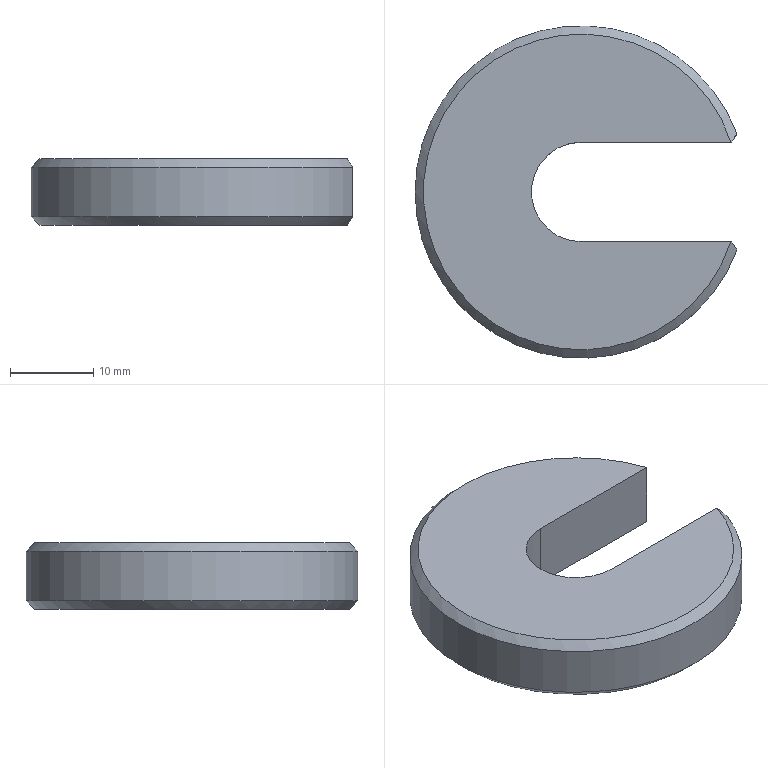Component | NX | SPLIT_WASHER | 1 solid | 10 faces | box 38.74 x 40 x 8 mm | volume 7592 mm3 | plane 6 | cylinder 2 | cone 2 | commonest cylinder face diameters 40 x1 12 x1
STEP:
#1=CARTESIAN_POINT('',(0.,0.,0.));
#2=DIRECTION('',(0.,0.,1.));
#3=DIRECTION('',(1.,0.,0.));
#4=AXIS2_PLACEMENT_3D('',#1,#2,#3);
#5=CARTESIAN_POINT('',(108.735,77.382,82.));
#6=VERTEX_POINT('',#5);
#7=CARTESIAN_POINT('',(108.735,77.382,76.));
#8=VERTEX_POINT('',#7);
#9=CARTESIAN_POINT('',(108.735,77.382,83.));
#10=DIRECTION('',(0.,0.,-1.));
#11=VECTOR('',#10,1.);
#12=LINE('',#9,#11);
#13=CARTESIAN_POINT('',(89.996,70.391,83.));
#14=DIRECTION('',(0.,0.,-1.));
#15=DIRECTION('',(-1.,0.,0.));
#16=AXIS2_PLACEMENT_3D('',#13,#14,#15);
#17=CYLINDRICAL_SURFACE('',#16,20.);
#18=CARTESIAN_POINT('',(2.785,0.));
#19=DIRECTION('',(0.,1.));
#20=VECTOR('',#19,1.);
#21=LINE('',#18,#20);
#22=(GEOMETRIC_REPRESENTATION_CONTEXT(2)PARAMETRIC_REPRESENTATION_CONTEXT()REPRESENTATION_CONTEXT('',''));
#23=DEFINITIONAL_REPRESENTATION('',(#21),#22);
#24=PCURVE('',#17,#23);
#25=CARTESIAN_POINT('',(108.735,77.382,83.));
#26=DIRECTION('',(-0.8214,0.5703,0.));
#27=DIRECTION('',(0.,0.,-1.));
#28=AXIS2_PLACEMENT_3D('',#25,#26,#27);
#29=PLANE('',#28);
#30=CARTESIAN_POINT('',(0.,0.));
#31=DIRECTION('',(1.,0.));
#32=VECTOR('',#31,1.);
#33=LINE('',#30,#32);
#34=(GEOMETRIC_REPRESENTATION_CONTEXT(2)PARAMETRIC_REPRESENTATION_CONTEXT()REPRESENTATION_CONTEXT('',''));
#35=DEFINITIONAL_REPRESENTATION('',(#33),#34);
#36=PCURVE('',#29,#35);
#37=SURFACE_CURVE('',#12,(#24,#36),.PCURVE_S1.);
#38=EDGE_CURVE('',#6,#8,#37,.T.);
#39=ORIENTED_EDGE('',*,*,#38,.T.);
#40=CARTESIAN_POINT('',(108.735,63.401,76.));
#41=VERTEX_POINT('',#40);
#42=CARTESIAN_POINT('',(89.996,70.391,76.));
#43=DIRECTION('',(0.,0.,1.));
#44=DIRECTION('',(1.,0.,0.));
#45=AXIS2_PLACEMENT_3D('',#42,#43,#44);
#46=CIRCLE('',#45,20.);
#47=CARTESIAN_POINT('',(3.142,7.));
#48=DIRECTION('',(-1.,0.));
#49=VECTOR('',#48,1.);
#50=LINE('',#47,#49);
#51=(GEOMETRIC_REPRESENTATION_CONTEXT(2)PARAMETRIC_REPRESENTATION_CONTEXT()REPRESENTATION_CONTEXT('',''));
#52=DEFINITIONAL_REPRESENTATION('',(#50),#51);
#53=PCURVE('',#17,#52);
#54=CARTESIAN_POINT('',(89.996,70.391,76.));
#55=DIRECTION('',(0.,0.,1.));
#56=DIRECTION('',(1.,0.,0.));
#57=AXIS2_PLACEMENT_3D('',#54,#55,#56);
#58=CONICAL_SURFACE('',#57,20.,0.7854);
#59=CARTESIAN_POINT('',(-0.,-0.));
#60=DIRECTION('',(1.,0.));
#61=VECTOR('',#60,1.);
#62=LINE('',#59,#61);
#63=(GEOMETRIC_REPRESENTATION_CONTEXT(2)PARAMETRIC_REPRESENTATION_CONTEXT()REPRESENTATION_CONTEXT('',''));
#64=DEFINITIONAL_REPRESENTATION('',(#62),#63);
#65=PCURVE('',#58,#64);
#66=SURFACE_CURVE('',#46,(#53,#65),.PCURVE_S1.);
#67=EDGE_CURVE('',#8,#41,#66,.T.);
#68=ORIENTED_EDGE('',*,*,#67,.T.);
#69=CARTESIAN_POINT('',(108.735,63.401,82.));
#70=VERTEX_POINT('',#69);
#71=CARTESIAN_POINT('',(108.735,63.401,83.));
#72=DIRECTION('',(0.,0.,1.));
#73=VECTOR('',#72,1.);
#74=LINE('',#71,#73);
#75=CARTESIAN_POINT('',(-2.785,0.));
#76=DIRECTION('',(0.,-1.));
#77=VECTOR('',#76,1.);
#78=LINE('',#75,#77);
#79=(GEOMETRIC_REPRESENTATION_CONTEXT(2)PARAMETRIC_REPRESENTATION_CONTEXT()REPRESENTATION_CONTEXT('',''));
#80=DEFINITIONAL_REPRESENTATION('',(#78),#79);
#81=PCURVE('',#17,#80);
#82=CARTESIAN_POINT('',(108.047,64.391,83.));
#83=DIRECTION('',(-0.8214,-0.5703,0.));
#84=DIRECTION('',(0.,0.,-1.));
#85=AXIS2_PLACEMENT_3D('',#82,#83,#84);
#86=PLANE('',#85);
#87=CARTESIAN_POINT('',(0.,1.206));
#88=DIRECTION('',(-1.,0.));
#89=VECTOR('',#88,1.);
#90=LINE('',#87,#89);
#91=(GEOMETRIC_REPRESENTATION_CONTEXT(2)PARAMETRIC_REPRESENTATION_CONTEXT()REPRESENTATION_CONTEXT('',''));
#92=DEFINITIONAL_REPRESENTATION('',(#90),#91);
#93=PCURVE('',#86,#92);
#94=SURFACE_CURVE('',#74,(#81,#93),.PCURVE_S1.);
#95=EDGE_CURVE('',#41,#70,#94,.T.);
#96=ORIENTED_EDGE('',*,*,#95,.T.);
#97=CARTESIAN_POINT('',(89.996,70.391,82.));
#98=DIRECTION('',(0.,0.,-1.));
#99=DIRECTION('',(1.,0.,0.));
#100=AXIS2_PLACEMENT_3D('',#97,#98,#99);
#101=CIRCLE('',#100,20.);
#102=CARTESIAN_POINT('',(-3.142,1.));
#103=DIRECTION('',(1.,0.));
#104=VECTOR('',#103,1.);
#105=LINE('',#102,#104);
#106=(GEOMETRIC_REPRESENTATION_CONTEXT(2)PARAMETRIC_REPRESENTATION_CONTEXT()REPRESENTATION_CONTEXT('',''));
#107=DEFINITIONAL_REPRESENTATION('',(#105),#106);
#108=PCURVE('',#17,#107);
#109=CARTESIAN_POINT('',(89.996,70.391,83.));
#110=DIRECTION('',(0.,0.,-1.));
#111=DIRECTION('',(-1.,0.,0.));
#112=AXIS2_PLACEMENT_3D('',#109,#110,#111);
#113=CONICAL_SURFACE('',#112,19.,0.7854);
#114=CARTESIAN_POINT('',(-3.142,1.));
#115=DIRECTION('',(1.,0.));
#116=VECTOR('',#115,1.);
#117=LINE('',#114,#116);
#118=(GEOMETRIC_REPRESENTATION_CONTEXT(2)PARAMETRIC_REPRESENTATION_CONTEXT()REPRESENTATION_CONTEXT('',''));
#119=DEFINITIONAL_REPRESENTATION('',(#117),#118);
#120=PCURVE('',#113,#119);
#121=SURFACE_CURVE('',#101,(#108,#120),.PCURVE_S1.);
#122=EDGE_CURVE('',#70,#6,#121,.T.);
#123=ORIENTED_EDGE('',*,*,#122,.T.);
#124=EDGE_LOOP('',(#39,#68,#96,#123));
#125=FACE_BOUND('',#124,.T.);
#126=ADVANCED_FACE('',(#125),#17,.T.);
#127=CARTESIAN_POINT('',(108.047,64.391,82.978));
#128=VERTEX_POINT('',#127);
#129=CARTESIAN_POINT('',(108.047,64.391,75.022));
#130=VERTEX_POINT('',#129);
#131=CARTESIAN_POINT('',(108.047,64.391,83.));
#132=DIRECTION('',(0.,0.,-1.));
#133=VECTOR('',#132,1.);
#134=LINE('',#131,#133);
#135=CARTESIAN_POINT('',(109.075,64.391,83.));
#136=DIRECTION('',(0.,-1.,0.));
#137=DIRECTION('',(0.,0.,-1.));
#138=AXIS2_PLACEMENT_3D('',#135,#136,#137);
#139=PLANE('',#138);
#140=CARTESIAN_POINT('',(0.,-1.028));
#141=DIRECTION('',(1.,0.));
#142=VECTOR('',#141,1.);
#143=LINE('',#140,#142);
#144=(GEOMETRIC_REPRESENTATION_CONTEXT(2)PARAMETRIC_REPRESENTATION_CONTEXT()REPRESENTATION_CONTEXT('',''));
#145=DEFINITIONAL_REPRESENTATION('',(#143),#144);
#146=PCURVE('',#139,#145);
#147=CARTESIAN_POINT('',(0.,0.));
#148=DIRECTION('',(1.,0.));
#149=VECTOR('',#148,1.);
#150=LINE('',#147,#149);
#151=(GEOMETRIC_REPRESENTATION_CONTEXT(2)PARAMETRIC_REPRESENTATION_CONTEXT()REPRESENTATION_CONTEXT('',''));
#152=DEFINITIONAL_REPRESENTATION('',(#150),#151);
#153=PCURVE('',#86,#152);
#154=SURFACE_CURVE('',#134,(#146,#153),.PCURVE_S1.);
#155=EDGE_CURVE('',#128,#130,#154,.T.);
#156=ORIENTED_EDGE('',*,*,#155,.T.);
#157=CARTESIAN_POINT('',(108.024,64.391,75.));
#158=VERTEX_POINT('',#157);
#159=CARTESIAN_POINT('',(108.047,64.391,75.022));
#160=CARTESIAN_POINT('',(108.039,64.391,75.015));
#161=CARTESIAN_POINT('',(108.031,64.391,75.007));
#162=CARTESIAN_POINT('',(108.024,64.391,75.));
#163=B_SPLINE_CURVE_WITH_KNOTS('',3,(#159,#160,#161,#162),.UNSPECIFIED.,.F.,.F.,(4,4),(0.,1.),.PIECEWISE_BEZIER_KNOTS.);
#164=CARTESIAN_POINT('',(7.978,-1.028));
#165=CARTESIAN_POINT('',(7.985,-1.035));
#166=CARTESIAN_POINT('',(7.993,-1.043));
#167=CARTESIAN_POINT('',(8.,-1.051));
#168=B_SPLINE_CURVE_WITH_KNOTS('',3,(#164,#165,#166,#167),.UNSPECIFIED.,.F.,.F.,(4,4),(0.,1.),.PIECEWISE_BEZIER_KNOTS.);
#169=(GEOMETRIC_REPRESENTATION_CONTEXT(2)PARAMETRIC_REPRESENTATION_CONTEXT()REPRESENTATION_CONTEXT('',''));
#170=DEFINITIONAL_REPRESENTATION('',(#168),#169);
#171=PCURVE('',#139,#170);
#172=CARTESIAN_POINT('',(5.962,-0.9778));
#173=CARTESIAN_POINT('',(5.962,-1.));
#174=B_SPLINE_CURVE_WITH_KNOTS('',1,(#172,#173),.UNSPECIFIED.,.F.,.F.,(2,2),(0.,1.),.PIECEWISE_BEZIER_KNOTS.);
#175=(GEOMETRIC_REPRESENTATION_CONTEXT(2)PARAMETRIC_REPRESENTATION_CONTEXT()REPRESENTATION_CONTEXT('',''));
#176=DEFINITIONAL_REPRESENTATION('',(#174),#175);
#177=PCURVE('',#58,#176);
#178=SURFACE_CURVE('',#163,(#171,#177),.PCURVE_S1.);
#179=EDGE_CURVE('',#130,#158,#178,.T.);
#180=ORIENTED_EDGE('',*,*,#179,.T.);
#181=CARTESIAN_POINT('',(89.996,64.391,75.));
#182=VERTEX_POINT('',#181);
#183=CARTESIAN_POINT('',(109.075,64.391,75.));
#184=DIRECTION('',(-1.,0.,0.));
#185=VECTOR('',#184,1.);
#186=LINE('',#183,#185);
#187=CARTESIAN_POINT('',(8.,0.));
#188=DIRECTION('',(0.,-1.));
#189=VECTOR('',#188,1.);
#190=LINE('',#187,#189);
#191=(GEOMETRIC_REPRESENTATION_CONTEXT(2)PARAMETRIC_REPRESENTATION_CONTEXT()REPRESENTATION_CONTEXT('',''));
#192=DEFINITIONAL_REPRESENTATION('',(#190),#191);
#193=PCURVE('',#139,#192);
#194=CARTESIAN_POINT('',(89.996,70.391,75.));
#195=DIRECTION('',(0.,0.,1.));
#196=DIRECTION('',(1.,0.,0.));
#197=AXIS2_PLACEMENT_3D('',#194,#195,#196);
#198=PLANE('',#197);
#199=CARTESIAN_POINT('',(19.079,-6.));
#200=DIRECTION('',(-1.,0.));
#201=VECTOR('',#200,1.);
#202=LINE('',#199,#201);
#203=(GEOMETRIC_REPRESENTATION_CONTEXT(2)PARAMETRIC_REPRESENTATION_CONTEXT()REPRESENTATION_CONTEXT('',''));
#204=DEFINITIONAL_REPRESENTATION('',(#202),#203);
#205=PCURVE('',#198,#204);
#206=SURFACE_CURVE('',#186,(#193,#205),.PCURVE_S1.);
#207=EDGE_CURVE('',#158,#182,#206,.T.);
#208=ORIENTED_EDGE('',*,*,#207,.T.);
#209=CARTESIAN_POINT('',(89.996,64.391,83.));
#210=VERTEX_POINT('',#209);
#211=CARTESIAN_POINT('',(89.996,64.391,83.));
#212=DIRECTION('',(0.,0.,-1.));
#213=VECTOR('',#212,1.);
#214=LINE('',#211,#213);
#215=CARTESIAN_POINT('',(0.,-19.079));
#216=DIRECTION('',(1.,0.));
#217=VECTOR('',#216,1.);
#218=LINE('',#215,#217);
#219=(GEOMETRIC_REPRESENTATION_CONTEXT(2)PARAMETRIC_REPRESENTATION_CONTEXT()REPRESENTATION_CONTEXT('',''));
#220=DEFINITIONAL_REPRESENTATION('',(#218),#219);
#221=PCURVE('',#139,#220);
#222=CARTESIAN_POINT('',(89.996,70.391,83.));
#223=DIRECTION('',(0.,0.,-1.));
#224=DIRECTION('',(-1.,0.,0.));
#225=AXIS2_PLACEMENT_3D('',#222,#223,#224);
#226=CYLINDRICAL_SURFACE('',#225,6.);
#227=CARTESIAN_POINT('',(-1.571,0.));
#228=DIRECTION('',(0.,1.));
#229=VECTOR('',#228,1.);
#230=LINE('',#227,#229);
#231=(GEOMETRIC_REPRESENTATION_CONTEXT(2)PARAMETRIC_REPRESENTATION_CONTEXT()REPRESENTATION_CONTEXT('',''));
#232=DEFINITIONAL_REPRESENTATION('',(#230),#231);
#233=PCURVE('',#226,#232);
#234=SURFACE_CURVE('',#214,(#221,#233),.PCURVE_S1.);
#235=EDGE_CURVE('',#210,#182,#234,.T.);
#236=ORIENTED_EDGE('',*,*,#235,.F.);
#237=CARTESIAN_POINT('',(108.024,64.391,83.));
#238=VERTEX_POINT('',#237);
#239=CARTESIAN_POINT('',(109.075,64.391,83.));
#240=DIRECTION('',(-1.,0.,0.));
#241=VECTOR('',#240,1.);
#242=LINE('',#239,#241);
#243=CARTESIAN_POINT('',(0.,0.));
#244=DIRECTION('',(0.,-1.));
#245=VECTOR('',#244,1.);
#246=LINE('',#243,#245);
#247=(GEOMETRIC_REPRESENTATION_CONTEXT(2)PARAMETRIC_REPRESENTATION_CONTEXT()REPRESENTATION_CONTEXT('',''));
#248=DEFINITIONAL_REPRESENTATION('',(#246),#247);
#249=PCURVE('',#139,#248);
#250=CARTESIAN_POINT('',(89.996,70.391,83.));
#251=DIRECTION('',(0.,0.,1.));
#252=DIRECTION('',(1.,0.,0.));
#253=AXIS2_PLACEMENT_3D('',#250,#251,#252);
#254=PLANE('',#253);
#255=CARTESIAN_POINT('',(19.079,-6.));
#256=DIRECTION('',(-1.,0.));
#257=VECTOR('',#256,1.);
#258=LINE('',#255,#257);
#259=(GEOMETRIC_REPRESENTATION_CONTEXT(2)PARAMETRIC_REPRESENTATION_CONTEXT()REPRESENTATION_CONTEXT('',''));
#260=DEFINITIONAL_REPRESENTATION('',(#258),#259);
#261=PCURVE('',#254,#260);
#262=SURFACE_CURVE('',#242,(#249,#261),.PCURVE_S1.);
#263=EDGE_CURVE('',#238,#210,#262,.T.);
#264=ORIENTED_EDGE('',*,*,#263,.F.);
#265=CARTESIAN_POINT('',(108.024,64.391,83.));
#266=CARTESIAN_POINT('',(108.031,64.391,82.993));
#267=CARTESIAN_POINT('',(108.039,64.391,82.985));
#268=CARTESIAN_POINT('',(108.047,64.391,82.978));
#269=B_SPLINE_CURVE_WITH_KNOTS('',3,(#265,#266,#267,#268),.UNSPECIFIED.,.F.,.F.,(4,4),(0.,1.),.PIECEWISE_BEZIER_KNOTS.);
#270=CARTESIAN_POINT('',(0.,-1.051));
#271=CARTESIAN_POINT('',(0.007385,-1.043));
#272=CARTESIAN_POINT('',(0.01477,-1.035));
#273=CARTESIAN_POINT('',(0.02216,-1.028));
#274=B_SPLINE_CURVE_WITH_KNOTS('',3,(#270,#271,#272,#273),.UNSPECIFIED.,.F.,.F.,(4,4),(0.,1.),.PIECEWISE_BEZIER_KNOTS.);
#275=(GEOMETRIC_REPRESENTATION_CONTEXT(2)PARAMETRIC_REPRESENTATION_CONTEXT()REPRESENTATION_CONTEXT('',''));
#276=DEFINITIONAL_REPRESENTATION('',(#274),#275);
#277=PCURVE('',#139,#276);
#278=CARTESIAN_POINT('',(-2.82,0.));
#279=CARTESIAN_POINT('',(-2.821,0.02216));
#280=B_SPLINE_CURVE_WITH_KNOTS('',1,(#278,#279),.UNSPECIFIED.,.F.,.F.,(2,2),(0.,1.),.PIECEWISE_BEZIER_KNOTS.);
#281=(GEOMETRIC_REPRESENTATION_CONTEXT(2)PARAMETRIC_REPRESENTATION_CONTEXT()REPRESENTATION_CONTEXT('',''));
#282=DEFINITIONAL_REPRESENTATION('',(#280),#281);
#283=PCURVE('',#113,#282);
#284=SURFACE_CURVE('',#269,(#277,#283),.PCURVE_S1.);
#285=EDGE_CURVE('',#238,#128,#284,.T.);
#286=ORIENTED_EDGE('',*,*,#285,.T.);
#287=EDGE_LOOP('',(#156,#180,#208,#236,#264,#286));
#288=FACE_BOUND('',#287,.T.);
#289=ADVANCED_FACE('',(#288),#139,.F.);
#290=ORIENTED_EDGE('',*,*,#235,.F.);
#291=CARTESIAN_POINT('',(89.996,76.391,83.));
#292=VERTEX_POINT('',#291);
#293=CARTESIAN_POINT('',(89.996,70.391,83.));
#294=DIRECTION('',(0.,0.,-1.));
#295=DIRECTION('',(1.,0.,0.));
#296=AXIS2_PLACEMENT_3D('',#293,#294,#295);
#297=CIRCLE('',#296,6.);
#298=CARTESIAN_POINT('',(-3.142,0.));
#299=DIRECTION('',(1.,0.));
#300=VECTOR('',#299,1.);
#301=LINE('',#298,#300);
#302=(GEOMETRIC_REPRESENTATION_CONTEXT(2)PARAMETRIC_REPRESENTATION_CONTEXT()REPRESENTATION_CONTEXT('',''));
#303=DEFINITIONAL_REPRESENTATION('',(#301),#302);
#304=PCURVE('',#226,#303);
#305=CARTESIAN_POINT('',(6.,0.));
#306=CARTESIAN_POINT('',(6.,-10.392));
#307=CARTESIAN_POINT('',(-3.,-5.196));
#308=CARTESIAN_POINT('',(-12.,-0.));
#309=CARTESIAN_POINT('',(-3.,5.196));
#310=CARTESIAN_POINT('',(6.,10.392));
#311=CARTESIAN_POINT('',(6.,0.));
#312=(BOUNDED_CURVE()B_SPLINE_CURVE(2,(#305,#306,#307,#308,#309,#310,#311),.UNSPECIFIED.,.T.,.F.)B_SPLINE_CURVE_WITH_KNOTS((1,2,2,2,2,1),(-2.094,0.,2.094,4.189,6.283,8.378),.UNSPECIFIED.)CURVE()GEOMETRIC_REPRESENTATION_ITEM()RATIONAL_B_SPLINE_CURVE((1.,0.5,1.,0.5,1.,0.5,1.))REPRESENTATION_ITEM(''));
#313=(GEOMETRIC_REPRESENTATION_CONTEXT(2)PARAMETRIC_REPRESENTATION_CONTEXT()REPRESENTATION_CONTEXT('',''));
#314=DEFINITIONAL_REPRESENTATION('',(#312),#313);
#315=PCURVE('',#254,#314);
#316=SURFACE_CURVE('',#297,(#304,#315),.PCURVE_S1.);
#317=EDGE_CURVE('',#210,#292,#316,.T.);
#318=ORIENTED_EDGE('',*,*,#317,.T.);
#319=CARTESIAN_POINT('',(89.996,76.391,75.));
#320=VERTEX_POINT('',#319);
#321=CARTESIAN_POINT('',(89.996,76.391,83.));
#322=DIRECTION('',(0.,0.,-1.));
#323=VECTOR('',#322,1.);
#324=LINE('',#321,#323);
#325=CARTESIAN_POINT('',(1.571,0.));
#326=DIRECTION('',(0.,1.));
#327=VECTOR('',#326,1.);
#328=LINE('',#325,#327);
#329=(GEOMETRIC_REPRESENTATION_CONTEXT(2)PARAMETRIC_REPRESENTATION_CONTEXT()REPRESENTATION_CONTEXT('',''));
#330=DEFINITIONAL_REPRESENTATION('',(#328),#329);
#331=PCURVE('',#226,#330);
#332=CARTESIAN_POINT('',(89.996,76.391,83.));
#333=DIRECTION('',(0.,1.,0.));
#334=DIRECTION('',(0.,0.,1.));
#335=AXIS2_PLACEMENT_3D('',#332,#333,#334);
#336=PLANE('',#335);
#337=CARTESIAN_POINT('',(0.,0.));
#338=DIRECTION('',(-1.,0.));
#339=VECTOR('',#338,1.);
#340=LINE('',#337,#339);
#341=(GEOMETRIC_REPRESENTATION_CONTEXT(2)PARAMETRIC_REPRESENTATION_CONTEXT()REPRESENTATION_CONTEXT('',''));
#342=DEFINITIONAL_REPRESENTATION('',(#340),#341);
#343=PCURVE('',#336,#342);
#344=SURFACE_CURVE('',#324,(#331,#343),.PCURVE_S1.);
#345=EDGE_CURVE('',#292,#320,#344,.T.);
#346=ORIENTED_EDGE('',*,*,#345,.T.);
#347=CARTESIAN_POINT('',(89.996,70.391,75.));
#348=DIRECTION('',(0.,0.,-1.));
#349=DIRECTION('',(1.,0.,0.));
#350=AXIS2_PLACEMENT_3D('',#347,#348,#349);
#351=CIRCLE('',#350,6.);
#352=CARTESIAN_POINT('',(-3.142,8.));
#353=DIRECTION('',(1.,0.));
#354=VECTOR('',#353,1.);
#355=LINE('',#352,#354);
#356=(GEOMETRIC_REPRESENTATION_CONTEXT(2)PARAMETRIC_REPRESENTATION_CONTEXT()REPRESENTATION_CONTEXT('',''));
#357=DEFINITIONAL_REPRESENTATION('',(#355),#356);
#358=PCURVE('',#226,#357);
#359=CARTESIAN_POINT('',(6.,0.));
#360=CARTESIAN_POINT('',(6.,-10.392));
#361=CARTESIAN_POINT('',(-3.,-5.196));
#362=CARTESIAN_POINT('',(-12.,-0.));
#363=CARTESIAN_POINT('',(-3.,5.196));
#364=CARTESIAN_POINT('',(6.,10.392));
#365=CARTESIAN_POINT('',(6.,0.));
#366=(BOUNDED_CURVE()B_SPLINE_CURVE(2,(#359,#360,#361,#362,#363,#364,#365),.UNSPECIFIED.,.T.,.F.)B_SPLINE_CURVE_WITH_KNOTS((1,2,2,2,2,1),(-2.094,0.,2.094,4.189,6.283,8.378),.UNSPECIFIED.)CURVE()GEOMETRIC_REPRESENTATION_ITEM()RATIONAL_B_SPLINE_CURVE((1.,0.5,1.,0.5,1.,0.5,1.))REPRESENTATION_ITEM(''));
#367=(GEOMETRIC_REPRESENTATION_CONTEXT(2)PARAMETRIC_REPRESENTATION_CONTEXT()REPRESENTATION_CONTEXT('',''));
#368=DEFINITIONAL_REPRESENTATION('',(#366),#367);
#369=PCURVE('',#198,#368);
#370=SURFACE_CURVE('',#351,(#358,#369),.PCURVE_S1.);
#371=EDGE_CURVE('',#182,#320,#370,.T.);
#372=ORIENTED_EDGE('',*,*,#371,.F.);
#373=EDGE_LOOP('',(#290,#318,#346,#372));
#374=FACE_BOUND('',#373,.F.);
#375=ADVANCED_FACE('',(#374),#226,.F.);
#376=CARTESIAN_POINT('',(108.024,76.391,75.));
#377=VERTEX_POINT('',#376);
#378=CARTESIAN_POINT('',(89.996,76.391,75.));
#379=DIRECTION('',(1.,0.,0.));
#380=VECTOR('',#379,1.);
#381=LINE('',#378,#380);
#382=CARTESIAN_POINT('',(-8.,0.));
#383=DIRECTION('',(0.,1.));
#384=VECTOR('',#383,1.);
#385=LINE('',#382,#384);
#386=(GEOMETRIC_REPRESENTATION_CONTEXT(2)PARAMETRIC_REPRESENTATION_CONTEXT()REPRESENTATION_CONTEXT('',''));
#387=DEFINITIONAL_REPRESENTATION('',(#385),#386);
#388=PCURVE('',#336,#387);
#389=CARTESIAN_POINT('',(0.,6.));
#390=DIRECTION('',(1.,0.));
#391=VECTOR('',#390,1.);
#392=LINE('',#389,#391);
#393=(GEOMETRIC_REPRESENTATION_CONTEXT(2)PARAMETRIC_REPRESENTATION_CONTEXT()REPRESENTATION_CONTEXT('',''));
#394=DEFINITIONAL_REPRESENTATION('',(#392),#393);
#395=PCURVE('',#198,#394);
#396=SURFACE_CURVE('',#381,(#388,#395),.PCURVE_S1.);
#397=EDGE_CURVE('',#320,#377,#396,.T.);
#398=ORIENTED_EDGE('',*,*,#397,.T.);
#399=CARTESIAN_POINT('',(108.047,76.391,75.022));
#400=VERTEX_POINT('',#399);
#401=CARTESIAN_POINT('',(108.024,76.391,75.));
#402=CARTESIAN_POINT('',(108.031,76.391,75.007));
#403=CARTESIAN_POINT('',(108.039,76.391,75.015));
#404=CARTESIAN_POINT('',(108.047,76.391,75.022));
#405=B_SPLINE_CURVE_WITH_KNOTS('',3,(#401,#402,#403,#404),.UNSPECIFIED.,.F.,.F.,(4,4),(0.,1.),.PIECEWISE_BEZIER_KNOTS.);
#406=CARTESIAN_POINT('',(-8.,18.028));
#407=CARTESIAN_POINT('',(-7.993,18.036));
#408=CARTESIAN_POINT('',(-7.985,18.043));
#409=CARTESIAN_POINT('',(-7.978,18.051));
#410=B_SPLINE_CURVE_WITH_KNOTS('',3,(#406,#407,#408,#409),.UNSPECIFIED.,.F.,.F.,(4,4),(0.,1.),.PIECEWISE_BEZIER_KNOTS.);
#411=(GEOMETRIC_REPRESENTATION_CONTEXT(2)PARAMETRIC_REPRESENTATION_CONTEXT()REPRESENTATION_CONTEXT('',''));
#412=DEFINITIONAL_REPRESENTATION('',(#410),#411);
#413=PCURVE('',#336,#412);
#414=CARTESIAN_POINT('',(0.3213,-1.));
#415=CARTESIAN_POINT('',(0.3209,-0.9778));
#416=B_SPLINE_CURVE_WITH_KNOTS('',1,(#414,#415),.UNSPECIFIED.,.F.,.F.,(2,2),(0.,1.),.PIECEWISE_BEZIER_KNOTS.);
#417=(GEOMETRIC_REPRESENTATION_CONTEXT(2)PARAMETRIC_REPRESENTATION_CONTEXT()REPRESENTATION_CONTEXT('',''));
#418=DEFINITIONAL_REPRESENTATION('',(#416),#417);
#419=PCURVE('',#58,#418);
#420=SURFACE_CURVE('',#405,(#413,#419),.PCURVE_S1.);
#421=EDGE_CURVE('',#377,#400,#420,.T.);
#422=ORIENTED_EDGE('',*,*,#421,.T.);
#423=CARTESIAN_POINT('',(108.047,76.391,82.978));
#424=VERTEX_POINT('',#423);
#425=CARTESIAN_POINT('',(108.047,76.391,83.));
#426=DIRECTION('',(0.,0.,1.));
#427=VECTOR('',#426,1.);
#428=LINE('',#425,#427);
#429=CARTESIAN_POINT('',(0.,18.051));
#430=DIRECTION('',(1.,0.));
#431=VECTOR('',#430,1.);
#432=LINE('',#429,#431);
#433=(GEOMETRIC_REPRESENTATION_CONTEXT(2)PARAMETRIC_REPRESENTATION_CONTEXT()REPRESENTATION_CONTEXT('',''));
#434=DEFINITIONAL_REPRESENTATION('',(#432),#433);
#435=PCURVE('',#336,#434);
#436=CARTESIAN_POINT('',(0.,1.206));
#437=DIRECTION('',(-1.,0.));
#438=VECTOR('',#437,1.);
#439=LINE('',#436,#438);
#440=(GEOMETRIC_REPRESENTATION_CONTEXT(2)PARAMETRIC_REPRESENTATION_CONTEXT()REPRESENTATION_CONTEXT('',''));
#441=DEFINITIONAL_REPRESENTATION('',(#439),#440);
#442=PCURVE('',#29,#441);
#443=SURFACE_CURVE('',#428,(#435,#442),.PCURVE_S1.);
#444=EDGE_CURVE('',#400,#424,#443,.T.);
#445=ORIENTED_EDGE('',*,*,#444,.T.);
#446=CARTESIAN_POINT('',(108.024,76.391,83.));
#447=VERTEX_POINT('',#446);
#448=CARTESIAN_POINT('',(108.047,76.391,82.978));
#449=CARTESIAN_POINT('',(108.039,76.391,82.985));
#450=CARTESIAN_POINT('',(108.031,76.391,82.993));
#451=CARTESIAN_POINT('',(108.024,76.391,83.));
#452=B_SPLINE_CURVE_WITH_KNOTS('',3,(#448,#449,#450,#451),.UNSPECIFIED.,.F.,.F.,(4,4),(0.,1.),.PIECEWISE_BEZIER_KNOTS.);
#453=CARTESIAN_POINT('',(-0.02216,18.051));
#454=CARTESIAN_POINT('',(-0.01477,18.043));
#455=CARTESIAN_POINT('',(-0.007385,18.036));
#456=CARTESIAN_POINT('',(0.,18.028));
#457=B_SPLINE_CURVE_WITH_KNOTS('',3,(#453,#454,#455,#456),.UNSPECIFIED.,.F.,.F.,(4,4),(0.,1.),.PIECEWISE_BEZIER_KNOTS.);
#458=(GEOMETRIC_REPRESENTATION_CONTEXT(2)PARAMETRIC_REPRESENTATION_CONTEXT()REPRESENTATION_CONTEXT('',''));
#459=DEFINITIONAL_REPRESENTATION('',(#457),#458);
#460=PCURVE('',#336,#459);
#461=CARTESIAN_POINT('',(2.821,0.02216));
#462=CARTESIAN_POINT('',(2.82,0.));
#463=B_SPLINE_CURVE_WITH_KNOTS('',1,(#461,#462),.UNSPECIFIED.,.F.,.F.,(2,2),(0.,1.),.PIECEWISE_BEZIER_KNOTS.);
#464=(GEOMETRIC_REPRESENTATION_CONTEXT(2)PARAMETRIC_REPRESENTATION_CONTEXT()REPRESENTATION_CONTEXT('',''));
#465=DEFINITIONAL_REPRESENTATION('',(#463),#464);
#466=PCURVE('',#113,#465);
#467=SURFACE_CURVE('',#452,(#460,#466),.PCURVE_S1.);
#468=EDGE_CURVE('',#424,#447,#467,.T.);
#469=ORIENTED_EDGE('',*,*,#468,.T.);
#470=CARTESIAN_POINT('',(89.996,76.391,83.));
#471=DIRECTION('',(1.,0.,0.));
#472=VECTOR('',#471,1.);
#473=LINE('',#470,#472);
#474=CARTESIAN_POINT('',(0.,0.));
#475=DIRECTION('',(0.,1.));
#476=VECTOR('',#475,1.);
#477=LINE('',#474,#476);
#478=(GEOMETRIC_REPRESENTATION_CONTEXT(2)PARAMETRIC_REPRESENTATION_CONTEXT()REPRESENTATION_CONTEXT('',''));
#479=DEFINITIONAL_REPRESENTATION('',(#477),#478);
#480=PCURVE('',#336,#479);
#481=CARTESIAN_POINT('',(0.,6.));
#482=DIRECTION('',(1.,0.));
#483=VECTOR('',#482,1.);
#484=LINE('',#481,#483);
#485=(GEOMETRIC_REPRESENTATION_CONTEXT(2)PARAMETRIC_REPRESENTATION_CONTEXT()REPRESENTATION_CONTEXT('',''));
#486=DEFINITIONAL_REPRESENTATION('',(#484),#485);
#487=PCURVE('',#254,#486);
#488=SURFACE_CURVE('',#473,(#480,#487),.PCURVE_S1.);
#489=EDGE_CURVE('',#292,#447,#488,.T.);
#490=ORIENTED_EDGE('',*,*,#489,.F.);
#491=ORIENTED_EDGE('',*,*,#345,.T.);
#492=EDGE_LOOP('',(#398,#422,#445,#469,#490,#491));
#493=FACE_BOUND('',#492,.T.);
#494=ADVANCED_FACE('',(#493),#336,.F.);
#495=ORIENTED_EDGE('',*,*,#489,.T.);
#496=CARTESIAN_POINT('',(89.996,70.391,83.));
#497=DIRECTION('',(0.,0.,1.));
#498=DIRECTION('',(1.,0.,0.));
#499=AXIS2_PLACEMENT_3D('',#496,#497,#498);
#500=CIRCLE('',#499,19.);
#501=CARTESIAN_POINT('',(0.,0.));
#502=DIRECTION('',(1.,0.));
#503=AXIS2_PLACEMENT_2D('',#501,#502);
#504=CIRCLE('',#503,19.);
#505=(GEOMETRIC_REPRESENTATION_CONTEXT(2)PARAMETRIC_REPRESENTATION_CONTEXT()REPRESENTATION_CONTEXT('',''));
#506=DEFINITIONAL_REPRESENTATION('',(#504),#505);
#507=PCURVE('',#254,#506);
#508=CARTESIAN_POINT('',(3.142,0.));
#509=DIRECTION('',(-1.,0.));
#510=VECTOR('',#509,1.);
#511=LINE('',#508,#510);
#512=(GEOMETRIC_REPRESENTATION_CONTEXT(2)PARAMETRIC_REPRESENTATION_CONTEXT()REPRESENTATION_CONTEXT('',''));
#513=DEFINITIONAL_REPRESENTATION('',(#511),#512);
#514=PCURVE('',#113,#513);
#515=SURFACE_CURVE('',#500,(#507,#514),.PCURVE_S1.);
#516=EDGE_CURVE('',#447,#238,#515,.T.);
#517=ORIENTED_EDGE('',*,*,#516,.T.);
#518=ORIENTED_EDGE('',*,*,#263,.T.);
#519=ORIENTED_EDGE('',*,*,#317,.T.);
#520=EDGE_LOOP('',(#495,#517,#518,#519));
#521=FACE_BOUND('',#520,.T.);
#522=ADVANCED_FACE('',(#521),#254,.T.);
#523=ORIENTED_EDGE('',*,*,#207,.F.);
#524=CARTESIAN_POINT('',(89.996,70.391,75.));
#525=DIRECTION('',(0.,0.,-1.));
#526=DIRECTION('',(1.,0.,0.));
#527=AXIS2_PLACEMENT_3D('',#524,#525,#526);
#528=CIRCLE('',#527,19.);
#529=CARTESIAN_POINT('',(19.,0.));
#530=CARTESIAN_POINT('',(19.,-32.909));
#531=CARTESIAN_POINT('',(-9.5,-16.454));
#532=CARTESIAN_POINT('',(-38.,-0.));
#533=CARTESIAN_POINT('',(-9.5,16.454));
#534=CARTESIAN_POINT('',(19.,32.909));
#535=CARTESIAN_POINT('',(19.,0.));
#536=(BOUNDED_CURVE()B_SPLINE_CURVE(2,(#529,#530,#531,#532,#533,#534,#535),.UNSPECIFIED.,.T.,.F.)B_SPLINE_CURVE_WITH_KNOTS((1,2,2,2,2,1),(-2.094,0.,2.094,4.189,6.283,8.378),.UNSPECIFIED.)CURVE()GEOMETRIC_REPRESENTATION_ITEM()RATIONAL_B_SPLINE_CURVE((1.,0.5,1.,0.5,1.,0.5,1.))REPRESENTATION_ITEM(''));
#537=(GEOMETRIC_REPRESENTATION_CONTEXT(2)PARAMETRIC_REPRESENTATION_CONTEXT()REPRESENTATION_CONTEXT('',''));
#538=DEFINITIONAL_REPRESENTATION('',(#536),#537);
#539=PCURVE('',#198,#538);
#540=CARTESIAN_POINT('',(6.283,-1.));
#541=DIRECTION('',(-1.,0.));
#542=VECTOR('',#541,1.);
#543=LINE('',#540,#542);
#544=(GEOMETRIC_REPRESENTATION_CONTEXT(2)PARAMETRIC_REPRESENTATION_CONTEXT()REPRESENTATION_CONTEXT('',''));
#545=DEFINITIONAL_REPRESENTATION('',(#543),#544);
#546=PCURVE('',#58,#545);
#547=SURFACE_CURVE('',#528,(#539,#546),.PCURVE_S1.);
#548=EDGE_CURVE('',#158,#377,#547,.T.);
#549=ORIENTED_EDGE('',*,*,#548,.T.);
#550=ORIENTED_EDGE('',*,*,#397,.F.);
#551=ORIENTED_EDGE('',*,*,#371,.F.);
#552=EDGE_LOOP('',(#523,#549,#550,#551));
#553=FACE_BOUND('',#552,.T.);
#554=ADVANCED_FACE('',(#553),#198,.F.);
#555=ORIENTED_EDGE('',*,*,#95,.F.);
#556=CARTESIAN_POINT('',(108.735,63.401,76.));
#557=CARTESIAN_POINT('',(108.507,63.73,75.672));
#558=CARTESIAN_POINT('',(108.277,64.06,75.345));
#559=CARTESIAN_POINT('',(108.047,64.391,75.022));
#560=B_SPLINE_CURVE_WITH_KNOTS('',3,(#556,#557,#558,#559),.UNSPECIFIED.,.F.,.F.,(4,4),(0.,1.),.PIECEWISE_BEZIER_KNOTS.);
#561=CARTESIAN_POINT('',(7.,1.206));
#562=CARTESIAN_POINT('',(7.328,0.8057));
#563=CARTESIAN_POINT('',(7.655,0.404));
#564=CARTESIAN_POINT('',(7.978,0.));
#565=B_SPLINE_CURVE_WITH_KNOTS('',3,(#561,#562,#563,#564),.UNSPECIFIED.,.F.,.F.,(4,4),(0.,1.),.PIECEWISE_BEZIER_KNOTS.);
#566=(GEOMETRIC_REPRESENTATION_CONTEXT(2)PARAMETRIC_REPRESENTATION_CONTEXT()REPRESENTATION_CONTEXT('',''));
#567=DEFINITIONAL_REPRESENTATION('',(#565),#566);
#568=PCURVE('',#86,#567);
#569=CARTESIAN_POINT('',(5.926,-0.));
#570=CARTESIAN_POINT('',(5.962,-0.9778));
#571=B_SPLINE_CURVE_WITH_KNOTS('',1,(#569,#570),.UNSPECIFIED.,.F.,.F.,(2,2),(0.,1.),.PIECEWISE_BEZIER_KNOTS.);
#572=(GEOMETRIC_REPRESENTATION_CONTEXT(2)PARAMETRIC_REPRESENTATION_CONTEXT()REPRESENTATION_CONTEXT('',''));
#573=DEFINITIONAL_REPRESENTATION('',(#571),#572);
#574=PCURVE('',#58,#573);
#575=SURFACE_CURVE('',#560,(#568,#574),.PCURVE_S1.);
#576=EDGE_CURVE('',#41,#130,#575,.T.);
#577=ORIENTED_EDGE('',*,*,#576,.T.);
#578=ORIENTED_EDGE('',*,*,#155,.F.);
#579=CARTESIAN_POINT('',(108.047,64.391,82.978));
#580=CARTESIAN_POINT('',(108.277,64.06,82.655));
#581=CARTESIAN_POINT('',(108.507,63.73,82.328));
#582=CARTESIAN_POINT('',(108.735,63.401,82.));
#583=B_SPLINE_CURVE_WITH_KNOTS('',3,(#579,#580,#581,#582),.UNSPECIFIED.,.F.,.F.,(4,4),(0.,1.),.PIECEWISE_BEZIER_KNOTS.);
#584=CARTESIAN_POINT('',(0.02216,0.));
#585=CARTESIAN_POINT('',(0.3455,0.404));
#586=CARTESIAN_POINT('',(0.6716,0.8057));
#587=CARTESIAN_POINT('',(1.,1.206));
#588=B_SPLINE_CURVE_WITH_KNOTS('',3,(#584,#585,#586,#587),.UNSPECIFIED.,.F.,.F.,(4,4),(0.,1.),.PIECEWISE_BEZIER_KNOTS.);
#589=(GEOMETRIC_REPRESENTATION_CONTEXT(2)PARAMETRIC_REPRESENTATION_CONTEXT()REPRESENTATION_CONTEXT('',''));
#590=DEFINITIONAL_REPRESENTATION('',(#588),#589);
#591=PCURVE('',#86,#590);
#592=CARTESIAN_POINT('',(-2.821,0.02216));
#593=CARTESIAN_POINT('',(-2.785,1.));
#594=B_SPLINE_CURVE_WITH_KNOTS('',1,(#592,#593),.UNSPECIFIED.,.F.,.F.,(2,2),(0.,1.),.PIECEWISE_BEZIER_KNOTS.);
#595=(GEOMETRIC_REPRESENTATION_CONTEXT(2)PARAMETRIC_REPRESENTATION_CONTEXT()REPRESENTATION_CONTEXT('',''));
#596=DEFINITIONAL_REPRESENTATION('',(#594),#595);
#597=PCURVE('',#113,#596);
#598=SURFACE_CURVE('',#583,(#591,#597),.PCURVE_S1.);
#599=EDGE_CURVE('',#128,#70,#598,.T.);
#600=ORIENTED_EDGE('',*,*,#599,.T.);
#601=EDGE_LOOP('',(#555,#577,#578,#600));
#602=FACE_BOUND('',#601,.T.);
#603=ADVANCED_FACE('',(#602),#86,.F.);
#604=ORIENTED_EDGE('',*,*,#444,.F.);
#605=CARTESIAN_POINT('',(108.047,76.391,75.022));
#606=CARTESIAN_POINT('',(108.277,76.723,75.345));
#607=CARTESIAN_POINT('',(108.507,77.053,75.672));
#608=CARTESIAN_POINT('',(108.735,77.382,76.));
#609=B_SPLINE_CURVE_WITH_KNOTS('',3,(#605,#606,#607,#608),.UNSPECIFIED.,.F.,.F.,(4,4),(0.,1.),.PIECEWISE_BEZIER_KNOTS.);
#610=CARTESIAN_POINT('',(7.978,1.206));
#611=CARTESIAN_POINT('',(7.655,0.8016));
#612=CARTESIAN_POINT('',(7.328,0.3998));
#613=CARTESIAN_POINT('',(7.,0.));
#614=B_SPLINE_CURVE_WITH_KNOTS('',3,(#610,#611,#612,#613),.UNSPECIFIED.,.F.,.F.,(4,4),(0.,1.),.PIECEWISE_BEZIER_KNOTS.);
#615=(GEOMETRIC_REPRESENTATION_CONTEXT(2)PARAMETRIC_REPRESENTATION_CONTEXT()REPRESENTATION_CONTEXT('',''));
#616=DEFINITIONAL_REPRESENTATION('',(#614),#615);
#617=PCURVE('',#29,#616);
#618=CARTESIAN_POINT('',(0.3209,-0.9778));
#619=CARTESIAN_POINT('',(0.3571,-0.));
#620=B_SPLINE_CURVE_WITH_KNOTS('',1,(#618,#619),.UNSPECIFIED.,.F.,.F.,(2,2),(0.,1.),.PIECEWISE_BEZIER_KNOTS.);
#621=(GEOMETRIC_REPRESENTATION_CONTEXT(2)PARAMETRIC_REPRESENTATION_CONTEXT()REPRESENTATION_CONTEXT('',''));
#622=DEFINITIONAL_REPRESENTATION('',(#620),#621);
#623=PCURVE('',#58,#622);
#624=SURFACE_CURVE('',#609,(#617,#623),.PCURVE_S1.);
#625=EDGE_CURVE('',#400,#8,#624,.T.);
#626=ORIENTED_EDGE('',*,*,#625,.T.);
#627=ORIENTED_EDGE('',*,*,#38,.F.);
#628=CARTESIAN_POINT('',(108.735,77.382,82.));
#629=CARTESIAN_POINT('',(108.507,77.053,82.328));
#630=CARTESIAN_POINT('',(108.277,76.723,82.655));
#631=CARTESIAN_POINT('',(108.047,76.391,82.978));
#632=B_SPLINE_CURVE_WITH_KNOTS('',3,(#628,#629,#630,#631),.UNSPECIFIED.,.F.,.F.,(4,4),(0.,1.),.PIECEWISE_BEZIER_KNOTS.);
#633=CARTESIAN_POINT('',(1.,0.));
#634=CARTESIAN_POINT('',(0.6716,0.3998));
#635=CARTESIAN_POINT('',(0.3455,0.8016));
#636=CARTESIAN_POINT('',(0.02216,1.206));
#637=B_SPLINE_CURVE_WITH_KNOTS('',3,(#633,#634,#635,#636),.UNSPECIFIED.,.F.,.F.,(4,4),(0.,1.),.PIECEWISE_BEZIER_KNOTS.);
#638=(GEOMETRIC_REPRESENTATION_CONTEXT(2)PARAMETRIC_REPRESENTATION_CONTEXT()REPRESENTATION_CONTEXT('',''));
#639=DEFINITIONAL_REPRESENTATION('',(#637),#638);
#640=PCURVE('',#29,#639);
#641=CARTESIAN_POINT('',(2.785,1.));
#642=CARTESIAN_POINT('',(2.821,0.02216));
#643=B_SPLINE_CURVE_WITH_KNOTS('',1,(#641,#642),.UNSPECIFIED.,.F.,.F.,(2,2),(0.,1.),.PIECEWISE_BEZIER_KNOTS.);
#644=(GEOMETRIC_REPRESENTATION_CONTEXT(2)PARAMETRIC_REPRESENTATION_CONTEXT()REPRESENTATION_CONTEXT('',''));
#645=DEFINITIONAL_REPRESENTATION('',(#643),#644);
#646=PCURVE('',#113,#645);
#647=SURFACE_CURVE('',#632,(#640,#646),.PCURVE_S1.);
#648=EDGE_CURVE('',#6,#424,#647,.T.);
#649=ORIENTED_EDGE('',*,*,#648,.T.);
#650=EDGE_LOOP('',(#604,#626,#627,#649));
#651=FACE_BOUND('',#650,.T.);
#652=ADVANCED_FACE('',(#651),#29,.F.);
#653=ORIENTED_EDGE('',*,*,#421,.F.);
#654=ORIENTED_EDGE('',*,*,#548,.F.);
#655=ORIENTED_EDGE('',*,*,#179,.F.);
#656=ORIENTED_EDGE('',*,*,#576,.F.);
#657=ORIENTED_EDGE('',*,*,#67,.F.);
#658=ORIENTED_EDGE('',*,*,#625,.F.);
#659=EDGE_LOOP('',(#653,#654,#655,#656,#657,#658));
#660=FACE_BOUND('',#659,.T.);
#661=ADVANCED_FACE('',(#660),#58,.T.);
#662=ORIENTED_EDGE('',*,*,#648,.F.);
#663=ORIENTED_EDGE('',*,*,#122,.F.);
#664=ORIENTED_EDGE('',*,*,#599,.F.);
#665=ORIENTED_EDGE('',*,*,#285,.F.);
#666=ORIENTED_EDGE('',*,*,#516,.F.);
#667=ORIENTED_EDGE('',*,*,#468,.F.);
#668=EDGE_LOOP('',(#662,#663,#664,#665,#666,#667));
#669=FACE_BOUND('',#668,.T.);
#670=ADVANCED_FACE('',(#669),#113,.T.);
#671=CLOSED_SHELL('',(#126,#289,#375,#494,#522,#554,#603,#652,#661,#670));
#672=MANIFOLD_SOLID_BREP('',#671);
#673=(LENGTH_UNIT()NAMED_UNIT(*)SI_UNIT(.MILLI.,.METRE.));
#674=UNCERTAINTY_MEASURE_WITH_UNIT(LENGTH_MEASURE(0.005),#673,'','');
#675=(NAMED_UNIT(*)PLANE_ANGLE_UNIT()SI_UNIT($,.RADIAN.));
#676=(NAMED_UNIT(*)SI_UNIT($,.STERADIAN.)SOLID_ANGLE_UNIT());
#677=(GEOMETRIC_REPRESENTATION_CONTEXT(3)GLOBAL_UNCERTAINTY_ASSIGNED_CONTEXT((#674))GLOBAL_UNIT_ASSIGNED_CONTEXT((#673,#675,#676))REPRESENTATION_CONTEXT('',''));
#678=ADVANCED_BREP_SHAPE_REPRESENTATION('',(#4,#672),#677);